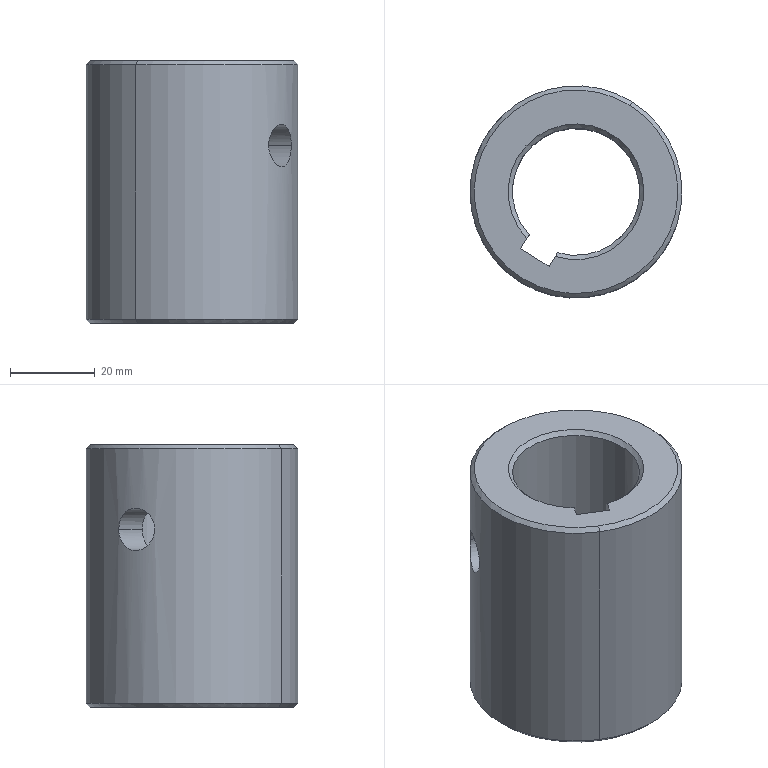Component | SolidWorks | 29-1 | 1 solid | 19 faces | box 50 x 50 x 62 mm | volume 74358 mm3 | cone 7 | cylinder 7 | plane 5 | commonest cylinder face diameters 10 x4 50 x2 30 x1
build123d program:
from build123d import *

# Parameters (mm, degrees)
SKETCH1_R           = 25
BOSS_EXTRUDE1_DEPTH = 31
SKETCH2_R           = 5
CUT_EXTRUDE1_DEPTH  = 31
CHAMFER1_SIZE       = 1
CHAMFER2_SIZE       = 1


with BuildPart() as part:
    # Sketch1 → Boss-Extrude1 (new, symmetric)
    with BuildSketch(Plane(origin=(0, 0, 0), x_dir=(1, 0, 0), z_dir=(0, 1, 0))):
        with Locations(Location((0, 0, 0), (0, 0, 270))):
            Circle(SKETCH1_R)
        with BuildLine():
            Line((4, 18.3), (-4, 18.3))
            Line((-4, 18.3), (-4, 14.457))
            ThreePointArc((-4, 14.457), (0, -15), (4, 14.457))
            Line((4, 14.457), (4, 18.3))
        make_face(mode=Mode.SUBTRACT)
    extrude(amount=BOSS_EXTRUDE1_DEPTH, both=True)

    # Sketch2 → Cut-Extrude1 (cut, symmetric)
    with BuildSketch(Plane(origin=(0, 0, 0), x_dir=(0, 0, -1), z_dir=(1, 0, 0))):
        with Locations((0, -11)):
            Circle(SKETCH2_R)
    extrude(amount=CUT_EXTRUDE1_DEPTH, both=True, mode=Mode.SUBTRACT)

    # Chamfer1
    chamfer1_edges = [part.edges().sort_by_distance(p)[0] for p in [
        (0, -31, 15),
        (0, 31, 15),
    ]]
    chamfer(chamfer1_edges, length=CHAMFER1_SIZE)

    # Chamfer2
    chamfer2_edges = [part.edges().sort_by_distance(p)[0] for p in [
        (0, -31, -25),
        (0, 31, -25),
    ]]
    chamfer(chamfer2_edges, length=CHAMFER2_SIZE)


solid = part.part

# Placed as in the assembly
solid = solid.moved(Location((70, -47, 137.06), (-89.999, 32.126, -0.0008769)))
STEP:
#1=CARTESIAN_POINT('',(2.253,-2.651,6.617));
#2=VERTEX_POINT('',#1);
#3=CARTESIAN_POINT('',(3.258,-1.05,6.617));
#4=VERTEX_POINT('',#3);
#5=CARTESIAN_POINT('',(2.756,-1.85,6.617));
#6=DIRECTION('',(0.,0.,1.));
#7=DIRECTION('',(0.5318,0.8469,0.));
#8=AXIS2_PLACEMENT_3D('',#5,#6,#7);
#9=CIRCLE('',#8,0.9449);
#10=EDGE_CURVE('',#2,#4,#9,.T.);
#11=ORIENTED_EDGE('',*,*,#10,.F.);
#12=CARTESIAN_POINT('',(2.232,-2.684,6.577));
#13=VERTEX_POINT('',#12);
#14=CARTESIAN_POINT('',(2.232,-2.684,6.577));
#15=DIRECTION('',(-0.376,-0.5988,-0.7071));
#16=VECTOR('',#15,39.37);
#17=LINE('',#14,#16);
#18=EDGE_CURVE('',#2,#13,#17,.T.);
#19=ORIENTED_EDGE('',*,*,#18,.T.);
#20=CARTESIAN_POINT('',(3.279,-1.017,6.577));
#21=VERTEX_POINT('',#20);
#22=CARTESIAN_POINT('',(2.756,-1.85,6.577));
#23=DIRECTION('',(-0.,-0.,-1.));
#24=DIRECTION('',(0.5318,0.8469,0.));
#25=AXIS2_PLACEMENT_3D('',#22,#23,#24);
#26=CIRCLE('',#25,0.9843);
#27=EDGE_CURVE('',#21,#13,#26,.T.);
#28=ORIENTED_EDGE('',*,*,#27,.F.);
#29=CARTESIAN_POINT('',(3.279,-1.017,6.577));
#30=DIRECTION('',(0.376,0.5988,-0.7071));
#31=VECTOR('',#30,39.37);
#32=LINE('',#29,#31);
#33=EDGE_CURVE('',#4,#21,#32,.T.);
#34=ORIENTED_EDGE('',*,*,#33,.F.);
#35=EDGE_LOOP('',(#11,#19,#28,#34));
#36=FACE_OUTER_BOUND('',#35,.T.);
#37=CARTESIAN_POINT('',(2.756,-1.85,6.577));
#38=DIRECTION('',(-0.,-0.,-1.));
#39=DIRECTION('',(0.5318,0.8469,0.));
#40=AXIS2_PLACEMENT_3D('',#37,#38,#39);
#41=CONICAL_SURFACE('',#40,0.9843,0.7854);
#42=ADVANCED_FACE('',(#36),#41,.T.);
#43=CARTESIAN_POINT('',(3.258,-1.05,4.176));
#44=VERTEX_POINT('',#43);
#45=CARTESIAN_POINT('',(2.253,-2.651,4.176));
#46=VERTEX_POINT('',#45);
#47=CARTESIAN_POINT('',(2.756,-1.85,4.176));
#48=DIRECTION('',(-0.,-0.,-1.));
#49=DIRECTION('',(0.5318,0.8469,0.));
#50=AXIS2_PLACEMENT_3D('',#47,#48,#49);
#51=CIRCLE('',#50,0.9449);
#52=EDGE_CURVE('',#44,#46,#51,.T.);
#53=ORIENTED_EDGE('',*,*,#52,.F.);
#54=CARTESIAN_POINT('',(3.279,-1.017,4.215));
#55=VERTEX_POINT('',#54);
#56=CARTESIAN_POINT('',(3.258,-1.05,4.176));
#57=DIRECTION('',(0.376,0.5988,0.7071));
#58=VECTOR('',#57,39.37);
#59=LINE('',#56,#58);
#60=EDGE_CURVE('',#44,#55,#59,.T.);
#61=ORIENTED_EDGE('',*,*,#60,.T.);
#62=CARTESIAN_POINT('',(2.232,-2.684,4.215));
#63=VERTEX_POINT('',#62);
#64=CARTESIAN_POINT('',(2.756,-1.85,4.215));
#65=DIRECTION('',(0.,0.,1.));
#66=DIRECTION('',(0.5318,0.8469,0.));
#67=AXIS2_PLACEMENT_3D('',#64,#65,#66);
#68=CIRCLE('',#67,0.9843);
#69=EDGE_CURVE('',#63,#55,#68,.T.);
#70=ORIENTED_EDGE('',*,*,#69,.F.);
#71=CARTESIAN_POINT('',(2.253,-2.651,4.176));
#72=DIRECTION('',(-0.376,-0.5988,0.7071));
#73=VECTOR('',#72,39.37);
#74=LINE('',#71,#73);
#75=EDGE_CURVE('',#46,#63,#74,.T.);
#76=ORIENTED_EDGE('',*,*,#75,.F.);
#77=EDGE_LOOP('',(#53,#61,#70,#76));
#78=FACE_OUTER_BOUND('',#77,.T.);
#79=CARTESIAN_POINT('',(2.756,-1.85,4.176));
#80=DIRECTION('',(0.,0.,1.));
#81=DIRECTION('',(-0.5318,-0.8469,0.));
#82=AXIS2_PLACEMENT_3D('',#79,#80,#81);
#83=CONICAL_SURFACE('',#82,0.9449,0.7854);
#84=ADVANCED_FACE('',(#78),#83,.T.);
#85=CARTESIAN_POINT('',(3.07,-1.35,4.215));
#86=VERTEX_POINT('',#85);
#87=CARTESIAN_POINT('',(2.587,-2.416,4.215));
#88=VERTEX_POINT('',#87);
#89=CARTESIAN_POINT('',(2.756,-1.85,4.215));
#90=DIRECTION('',(-0.,-0.,-1.));
#91=DIRECTION('',(0.5318,0.8469,0.));
#92=AXIS2_PLACEMENT_3D('',#89,#90,#91);
#93=CIRCLE('',#92,0.5906);
#94=EDGE_CURVE('',#86,#88,#93,.T.);
#95=ORIENTED_EDGE('',*,*,#94,.F.);
#96=CARTESIAN_POINT('',(3.091,-1.317,4.176));
#97=VERTEX_POINT('',#96);
#98=CARTESIAN_POINT('',(3.07,-1.35,4.215));
#99=DIRECTION('',(0.376,0.5988,-0.7071));
#100=VECTOR('',#99,39.37);
#101=LINE('',#98,#100);
#102=EDGE_CURVE('',#86,#97,#101,.T.);
#103=ORIENTED_EDGE('',*,*,#102,.T.);
#104=CARTESIAN_POINT('',(2.565,-2.451,4.176));
#105=VERTEX_POINT('',#104);
#106=CARTESIAN_POINT('',(2.756,-1.85,4.176));
#107=DIRECTION('',(0.,0.,1.));
#108=DIRECTION('',(0.5318,0.8469,0.));
#109=AXIS2_PLACEMENT_3D('',#106,#107,#108);
#110=CIRCLE('',#109,0.6299);
#111=EDGE_CURVE('',#105,#97,#110,.T.);
#112=ORIENTED_EDGE('',*,*,#111,.F.);
#113=CARTESIAN_POINT('',(2.587,-2.416,4.215));
#114=CARTESIAN_POINT('',(2.579,-2.428,4.202));
#115=CARTESIAN_POINT('',(2.572,-2.439,4.189));
#116=CARTESIAN_POINT('',(2.565,-2.451,4.176));
#117=B_SPLINE_CURVE_WITH_KNOTS('',3,(#113,#114,#115,#116),.UNSPECIFIED.,.F.,.F.,(4,4),(0.,0.001439),.UNSPECIFIED.);
#118=EDGE_CURVE('',#88,#105,#117,.T.);
#119=ORIENTED_EDGE('',*,*,#118,.F.);
#120=EDGE_LOOP('',(#95,#103,#112,#119));
#121=FACE_OUTER_BOUND('',#120,.T.);
#122=CARTESIAN_POINT('',(2.756,-1.85,4.215));
#123=DIRECTION('',(-0.,-0.,-1.));
#124=DIRECTION('',(0.5318,0.8469,0.));
#125=AXIS2_PLACEMENT_3D('',#122,#123,#124);
#126=CONICAL_SURFACE('',#125,0.5906,0.7854);
#127=ADVANCED_FACE('',(#121),#126,.F.);
#128=CARTESIAN_POINT('',(2.044,-1.171,5.829));
#129=VERTEX_POINT('',#128);
#130=CARTESIAN_POINT('',(1.835,-1.504,5.829));
#131=VERTEX_POINT('',#130);
#132=CARTESIAN_POINT('',(2.044,-1.171,5.829));
#133=CARTESIAN_POINT('',(2.044,-1.171,5.842));
#134=CARTESIAN_POINT('',(2.043,-1.172,5.855));
#135=CARTESIAN_POINT('',(2.039,-1.176,5.88));
#136=CARTESIAN_POINT('',(2.037,-1.178,5.893));
#137=CARTESIAN_POINT('',(2.032,-1.184,5.91));
#138=CARTESIAN_POINT('',(2.03,-1.186,5.916));
#139=CARTESIAN_POINT('',(2.026,-1.19,5.928));
#140=CARTESIAN_POINT('',(2.023,-1.193,5.933));
#141=CARTESIAN_POINT('',(2.016,-1.201,5.949));
#142=CARTESIAN_POINT('',(2.011,-1.207,5.959));
#143=CARTESIAN_POINT('',(1.999,-1.221,5.977));
#144=CARTESIAN_POINT('',(1.992,-1.229,5.986));
#145=CARTESIAN_POINT('',(1.979,-1.246,6.));
#146=CARTESIAN_POINT('',(1.972,-1.255,6.006));
#147=CARTESIAN_POINT('',(1.958,-1.274,6.016));
#148=CARTESIAN_POINT('',(1.951,-1.284,6.02));
#149=CARTESIAN_POINT('',(1.936,-1.305,6.025));
#150=CARTESIAN_POINT('',(1.929,-1.316,6.026));
#151=CARTESIAN_POINT('',(1.916,-1.338,6.026));
#152=CARTESIAN_POINT('',(1.909,-1.349,6.025));
#153=CARTESIAN_POINT('',(1.896,-1.371,6.02));
#154=CARTESIAN_POINT('',(1.89,-1.382,6.016));
#155=CARTESIAN_POINT('',(1.879,-1.403,6.006));
#156=CARTESIAN_POINT('',(1.874,-1.413,6.));
#157=CARTESIAN_POINT('',(1.867,-1.428,5.989));
#158=CARTESIAN_POINT('',(1.865,-1.432,5.985));
#159=CARTESIAN_POINT('',(1.861,-1.442,5.977));
#160=CARTESIAN_POINT('',(1.859,-1.446,5.973));
#161=CARTESIAN_POINT('',(1.853,-1.458,5.959));
#162=CARTESIAN_POINT('',(1.85,-1.466,5.949));
#163=CARTESIAN_POINT('',(1.844,-1.48,5.928));
#164=CARTESIAN_POINT('',(1.842,-1.485,5.917));
#165=CARTESIAN_POINT('',(1.838,-1.495,5.893));
#166=CARTESIAN_POINT('',(1.837,-1.498,5.88));
#167=CARTESIAN_POINT('',(1.835,-1.503,5.855));
#168=CARTESIAN_POINT('',(1.835,-1.504,5.842));
#169=CARTESIAN_POINT('',(1.835,-1.504,5.829));
#170=B_SPLINE_CURVE_WITH_KNOTS('',3,(#132,#133,#134,#135,#136,#137,#138,#139,#140,#141,#142,#143,#144,#145,#146,#147,#148,#149,#150,#151,#152,#153,#154,#155,#156,#157,#158,#159,#160,#161,#162,#163,#164,#165,#166,#167,#168,#169),.UNSPECIFIED.,.F.,.F.,(4,2,2,2,2,2,2,2,2,2,2,2,2,2,2,2,2,2,4),(0.01567,0.01665,0.01763,0.01812,0.01861,0.01959,0.02057,0.02155,0.02253,0.02351,0.02448,0.02546,0.02644,0.02693,0.02742,0.0284,0.02938,0.03036,0.03134),.UNSPECIFIED.);
#171=EDGE_CURVE('',#129,#131,#170,.T.);
#172=ORIENTED_EDGE('',*,*,#171,.F.);
#173=CARTESIAN_POINT('',(2.389,-1.388,5.829));
#174=VERTEX_POINT('',#173);
#175=CARTESIAN_POINT('',(1.827,-1.035,5.829));
#176=DIRECTION('',(0.8469,-0.5318,-0.));
#177=VECTOR('',#176,39.37);
#178=LINE('',#175,#177);
#179=EDGE_CURVE('',#129,#174,#178,.T.);
#180=ORIENTED_EDGE('',*,*,#179,.T.);
#181=CARTESIAN_POINT('',(2.18,-1.721,5.829));
#182=VERTEX_POINT('',#181);
#183=CARTESIAN_POINT('',(2.389,-1.388,5.829));
#184=CARTESIAN_POINT('',(2.389,-1.388,5.842));
#185=CARTESIAN_POINT('',(2.388,-1.388,5.855));
#186=CARTESIAN_POINT('',(2.384,-1.392,5.881));
#187=CARTESIAN_POINT('',(2.381,-1.394,5.893));
#188=CARTESIAN_POINT('',(2.373,-1.401,5.917));
#189=CARTESIAN_POINT('',(2.368,-1.405,5.928));
#190=CARTESIAN_POINT('',(2.357,-1.415,5.949));
#191=CARTESIAN_POINT('',(2.351,-1.421,5.959));
#192=CARTESIAN_POINT('',(2.337,-1.434,5.977));
#193=CARTESIAN_POINT('',(2.33,-1.441,5.986));
#194=CARTESIAN_POINT('',(2.315,-1.457,6.));
#195=CARTESIAN_POINT('',(2.308,-1.466,6.006));
#196=CARTESIAN_POINT('',(2.292,-1.484,6.016));
#197=CARTESIAN_POINT('',(2.285,-1.494,6.02));
#198=CARTESIAN_POINT('',(2.27,-1.514,6.025));
#199=CARTESIAN_POINT('',(2.263,-1.525,6.026));
#200=CARTESIAN_POINT('',(2.249,-1.547,6.026));
#201=CARTESIAN_POINT('',(2.242,-1.558,6.025));
#202=CARTESIAN_POINT('',(2.233,-1.575,6.021));
#203=CARTESIAN_POINT('',(2.23,-1.581,6.019));
#204=CARTESIAN_POINT('',(2.225,-1.592,6.016));
#205=CARTESIAN_POINT('',(2.222,-1.598,6.013));
#206=CARTESIAN_POINT('',(2.215,-1.614,6.006));
#207=CARTESIAN_POINT('',(2.21,-1.624,6.));
#208=CARTESIAN_POINT('',(2.202,-1.645,5.985));
#209=CARTESIAN_POINT('',(2.199,-1.654,5.977));
#210=CARTESIAN_POINT('',(2.193,-1.672,5.959));
#211=CARTESIAN_POINT('',(2.19,-1.68,5.949));
#212=CARTESIAN_POINT('',(2.186,-1.694,5.928));
#213=CARTESIAN_POINT('',(2.185,-1.7,5.917));
#214=CARTESIAN_POINT('',(2.182,-1.711,5.893));
#215=CARTESIAN_POINT('',(2.181,-1.714,5.88));
#216=CARTESIAN_POINT('',(2.18,-1.72,5.855));
#217=CARTESIAN_POINT('',(2.18,-1.721,5.842));
#218=CARTESIAN_POINT('',(2.18,-1.721,5.829));
#219=B_SPLINE_CURVE_WITH_KNOTS('',3,(#183,#184,#185,#186,#187,#188,#189,#190,#191,#192,#193,#194,#195,#196,#197,#198,#199,#200,#201,#202,#203,#204,#205,#206,#207,#208,#209,#210,#211,#212,#213,#214,#215,#216,#217,#218),.UNSPECIFIED.,.F.,.F.,(4,2,2,2,2,2,2,2,2,2,2,2,2,2,2,2,2,4),(0.01575,0.01673,0.01771,0.0187,0.01968,0.02066,0.02165,0.02263,0.02362,0.0246,0.02509,0.02558,0.02657,0.02755,0.02854,0.02952,0.0305,0.03149),.UNSPECIFIED.);
#220=EDGE_CURVE('',#174,#182,#219,.T.);
#221=ORIENTED_EDGE('',*,*,#220,.T.);
#222=CARTESIAN_POINT('',(1.618,-1.368,5.829));
#223=DIRECTION('',(0.8469,-0.5318,-0.));
#224=VECTOR('',#223,39.37);
#225=LINE('',#222,#224);
#226=EDGE_CURVE('',#131,#182,#225,.T.);
#227=ORIENTED_EDGE('',*,*,#226,.F.);
#228=EDGE_LOOP('',(#172,#180,#221,#227));
#229=FACE_OUTER_BOUND('',#228,.T.);
#230=CARTESIAN_POINT('',(1.722,-1.201,5.829));
#231=DIRECTION('',(0.8469,-0.5318,-0.));
#232=DIRECTION('',(-0.5318,-0.8469,0.));
#233=AXIS2_PLACEMENT_3D('',#230,#231,#232);
#234=CYLINDRICAL_SURFACE('',#233,0.1969);
#235=ADVANCED_FACE('',(#229),#234,.F.);
#236=CARTESIAN_POINT('',(3.123,-2.313,5.829));
#237=VERTEX_POINT('',#236);
#238=CARTESIAN_POINT('',(3.332,-1.98,5.829));
#239=VERTEX_POINT('',#238);
#240=CARTESIAN_POINT('',(3.123,-2.313,5.829));
#241=CARTESIAN_POINT('',(3.123,-2.313,5.842));
#242=CARTESIAN_POINT('',(3.124,-2.312,5.855));
#243=CARTESIAN_POINT('',(3.128,-2.309,5.88));
#244=CARTESIAN_POINT('',(3.131,-2.306,5.893));
#245=CARTESIAN_POINT('',(3.139,-2.3,5.917));
#246=CARTESIAN_POINT('',(3.144,-2.296,5.928));
#247=CARTESIAN_POINT('',(3.155,-2.286,5.949));
#248=CARTESIAN_POINT('',(3.161,-2.28,5.959));
#249=CARTESIAN_POINT('',(3.175,-2.267,5.977));
#250=CARTESIAN_POINT('',(3.182,-2.26,5.985));
#251=CARTESIAN_POINT('',(3.197,-2.244,6.));
#252=CARTESIAN_POINT('',(3.204,-2.235,6.006));
#253=CARTESIAN_POINT('',(3.215,-2.221,6.013));
#254=CARTESIAN_POINT('',(3.219,-2.217,6.015));
#255=CARTESIAN_POINT('',(3.227,-2.207,6.019));
#256=CARTESIAN_POINT('',(3.231,-2.202,6.021));
#257=CARTESIAN_POINT('',(3.242,-2.186,6.025));
#258=CARTESIAN_POINT('',(3.249,-2.175,6.026));
#259=CARTESIAN_POINT('',(3.263,-2.154,6.026));
#260=CARTESIAN_POINT('',(3.269,-2.142,6.025));
#261=CARTESIAN_POINT('',(3.282,-2.12,6.02));
#262=CARTESIAN_POINT('',(3.287,-2.109,6.016));
#263=CARTESIAN_POINT('',(3.297,-2.087,6.006));
#264=CARTESIAN_POINT('',(3.302,-2.076,6.));
#265=CARTESIAN_POINT('',(3.31,-2.056,5.986));
#266=CARTESIAN_POINT('',(3.313,-2.046,5.977));
#267=CARTESIAN_POINT('',(3.319,-2.029,5.959));
#268=CARTESIAN_POINT('',(3.321,-2.021,5.949));
#269=CARTESIAN_POINT('',(3.325,-2.007,5.928));
#270=CARTESIAN_POINT('',(3.327,-2.,5.917));
#271=CARTESIAN_POINT('',(3.33,-1.99,5.893));
#272=CARTESIAN_POINT('',(3.331,-1.986,5.881));
#273=CARTESIAN_POINT('',(3.332,-1.982,5.861));
#274=CARTESIAN_POINT('',(3.332,-1.981,5.855));
#275=CARTESIAN_POINT('',(3.332,-1.98,5.842));
#276=CARTESIAN_POINT('',(3.332,-1.98,5.836));
#277=CARTESIAN_POINT('',(3.332,-1.98,5.829));
#278=B_SPLINE_CURVE_WITH_KNOTS('',3,(#240,#241,#242,#243,#244,#245,#246,#247,#248,#249,#250,#251,#252,#253,#254,#255,#256,#257,#258,#259,#260,#261,#262,#263,#264,#265,#266,#267,#268,#269,#270,#271,#272,#273,#274,#275,#276,#277),.UNSPECIFIED.,.F.,.F.,(4,2,2,2,2,2,2,2,2,2,2,2,2,2,2,2,2,2,4),(0.,0.0009841,0.001968,0.002952,0.003936,0.00492,0.005905,0.006397,0.006889,0.007873,0.008857,0.009841,0.01082,0.01181,0.01279,0.01378,0.01476,0.01525,0.01575),.UNSPECIFIED.);
#279=EDGE_CURVE('',#237,#239,#278,.T.);
#280=ORIENTED_EDGE('',*,*,#279,.T.);
#281=CARTESIAN_POINT('',(3.677,-2.197,5.829));
#282=VERTEX_POINT('',#281);
#283=CARTESIAN_POINT('',(1.827,-1.035,5.829));
#284=DIRECTION('',(0.8469,-0.5318,-0.));
#285=VECTOR('',#284,39.37);
#286=LINE('',#283,#285);
#287=EDGE_CURVE('',#239,#282,#286,.T.);
#288=ORIENTED_EDGE('',*,*,#287,.T.);
#289=CARTESIAN_POINT('',(3.468,-2.53,5.829));
#290=VERTEX_POINT('',#289);
#291=CARTESIAN_POINT('',(3.468,-2.53,5.829));
#292=CARTESIAN_POINT('',(3.468,-2.53,5.842));
#293=CARTESIAN_POINT('',(3.469,-2.529,5.855));
#294=CARTESIAN_POINT('',(3.472,-2.525,5.88));
#295=CARTESIAN_POINT('',(3.475,-2.522,5.893));
#296=CARTESIAN_POINT('',(3.482,-2.515,5.917));
#297=CARTESIAN_POINT('',(3.486,-2.511,5.928));
#298=CARTESIAN_POINT('',(3.496,-2.5,5.949));
#299=CARTESIAN_POINT('',(3.501,-2.493,5.959));
#300=CARTESIAN_POINT('',(3.513,-2.479,5.977));
#301=CARTESIAN_POINT('',(3.519,-2.472,5.986));
#302=CARTESIAN_POINT('',(3.533,-2.455,6.));
#303=CARTESIAN_POINT('',(3.54,-2.446,6.006));
#304=CARTESIAN_POINT('',(3.554,-2.427,6.016));
#305=CARTESIAN_POINT('',(3.561,-2.416,6.02));
#306=CARTESIAN_POINT('',(3.576,-2.395,6.025));
#307=CARTESIAN_POINT('',(3.583,-2.385,6.026));
#308=CARTESIAN_POINT('',(3.596,-2.363,6.026));
#309=CARTESIAN_POINT('',(3.603,-2.352,6.025));
#310=CARTESIAN_POINT('',(3.616,-2.33,6.02));
#311=CARTESIAN_POINT('',(3.622,-2.319,6.016));
#312=CARTESIAN_POINT('',(3.63,-2.303,6.008));
#313=CARTESIAN_POINT('',(3.633,-2.298,6.006));
#314=CARTESIAN_POINT('',(3.638,-2.288,6.));
#315=CARTESIAN_POINT('',(3.64,-2.283,5.996));
#316=CARTESIAN_POINT('',(3.647,-2.268,5.986));
#317=CARTESIAN_POINT('',(3.651,-2.259,5.977));
#318=CARTESIAN_POINT('',(3.659,-2.242,5.959));
#319=CARTESIAN_POINT('',(3.662,-2.235,5.949));
#320=CARTESIAN_POINT('',(3.668,-2.221,5.928));
#321=CARTESIAN_POINT('',(3.67,-2.215,5.916));
#322=CARTESIAN_POINT('',(3.674,-2.206,5.893));
#323=CARTESIAN_POINT('',(3.675,-2.203,5.88));
#324=CARTESIAN_POINT('',(3.677,-2.198,5.855));
#325=CARTESIAN_POINT('',(3.677,-2.197,5.842));
#326=CARTESIAN_POINT('',(3.677,-2.197,5.829));
#327=B_SPLINE_CURVE_WITH_KNOTS('',3,(#291,#292,#293,#294,#295,#296,#297,#298,#299,#300,#301,#302,#303,#304,#305,#306,#307,#308,#309,#310,#311,#312,#313,#314,#315,#316,#317,#318,#319,#320,#321,#322,#323,#324,#325,#326),.UNSPECIFIED.,.F.,.F.,(4,2,2,2,2,2,2,2,2,2,2,2,2,2,2,2,2,4),(0.,0.0009795,0.001959,0.002938,0.003918,0.004897,0.005877,0.006856,0.007836,0.008815,0.009795,0.01028,0.01077,0.01175,0.01273,0.01371,0.01469,0.01567),.UNSPECIFIED.);
#328=EDGE_CURVE('',#290,#282,#327,.T.);
#329=ORIENTED_EDGE('',*,*,#328,.F.);
#330=CARTESIAN_POINT('',(1.618,-1.368,5.829));
#331=DIRECTION('',(0.8469,-0.5318,-0.));
#332=VECTOR('',#331,39.37);
#333=LINE('',#330,#332);
#334=EDGE_CURVE('',#237,#290,#333,.T.);
#335=ORIENTED_EDGE('',*,*,#334,.F.);
#336=EDGE_LOOP('',(#280,#288,#329,#335));
#337=FACE_OUTER_BOUND('',#336,.T.);
#338=CARTESIAN_POINT('',(1.722,-1.201,5.829));
#339=DIRECTION('',(0.8469,-0.5318,-0.));
#340=DIRECTION('',(-0.5318,-0.8469,0.));
#341=AXIS2_PLACEMENT_3D('',#338,#339,#340);
#342=CYLINDRICAL_SURFACE('',#341,0.1969);
#343=ADVANCED_FACE('',(#337),#342,.F.);
#344=ORIENTED_EDGE('',*,*,#328,.T.);
#345=CARTESIAN_POINT('',(3.677,-2.197,5.829));
#346=CARTESIAN_POINT('',(3.677,-2.197,5.816));
#347=CARTESIAN_POINT('',(3.677,-2.198,5.803));
#348=CARTESIAN_POINT('',(3.675,-2.203,5.778));
#349=CARTESIAN_POINT('',(3.674,-2.206,5.766));
#350=CARTESIAN_POINT('',(3.671,-2.213,5.748));
#351=CARTESIAN_POINT('',(3.67,-2.216,5.742));
#352=CARTESIAN_POINT('',(3.668,-2.221,5.731));
#353=CARTESIAN_POINT('',(3.666,-2.225,5.725));
#354=CARTESIAN_POINT('',(3.662,-2.235,5.709));
#355=CARTESIAN_POINT('',(3.659,-2.242,5.699));
#356=CARTESIAN_POINT('',(3.651,-2.259,5.681));
#357=CARTESIAN_POINT('',(3.647,-2.268,5.673));
#358=CARTESIAN_POINT('',(3.638,-2.288,5.658));
#359=CARTESIAN_POINT('',(3.633,-2.298,5.652));
#360=CARTESIAN_POINT('',(3.622,-2.319,5.642));
#361=CARTESIAN_POINT('',(3.616,-2.33,5.639));
#362=CARTESIAN_POINT('',(3.603,-2.352,5.634));
#363=CARTESIAN_POINT('',(3.596,-2.363,5.632));
#364=CARTESIAN_POINT('',(3.583,-2.385,5.632));
#365=CARTESIAN_POINT('',(3.576,-2.395,5.634));
#366=CARTESIAN_POINT('',(3.561,-2.416,5.639));
#367=CARTESIAN_POINT('',(3.554,-2.427,5.642));
#368=CARTESIAN_POINT('',(3.54,-2.446,5.652));
#369=CARTESIAN_POINT('',(3.533,-2.455,5.658));
#370=CARTESIAN_POINT('',(3.523,-2.467,5.669));
#371=CARTESIAN_POINT('',(3.52,-2.471,5.673));
#372=CARTESIAN_POINT('',(3.513,-2.479,5.681));
#373=CARTESIAN_POINT('',(3.51,-2.483,5.685));
#374=CARTESIAN_POINT('',(3.501,-2.493,5.699));
#375=CARTESIAN_POINT('',(3.496,-2.5,5.709));
#376=CARTESIAN_POINT('',(3.486,-2.51,5.73));
#377=CARTESIAN_POINT('',(3.482,-2.515,5.742));
#378=CARTESIAN_POINT('',(3.475,-2.522,5.765));
#379=CARTESIAN_POINT('',(3.472,-2.525,5.778));
#380=CARTESIAN_POINT('',(3.469,-2.529,5.803));
#381=CARTESIAN_POINT('',(3.468,-2.53,5.816));
#382=CARTESIAN_POINT('',(3.468,-2.53,5.829));
#383=B_SPLINE_CURVE_WITH_KNOTS('',3,(#345,#346,#347,#348,#349,#350,#351,#352,#353,#354,#355,#356,#357,#358,#359,#360,#361,#362,#363,#364,#365,#366,#367,#368,#369,#370,#371,#372,#373,#374,#375,#376,#377,#378,#379,#380,#381,#382),.UNSPECIFIED.,.F.,.F.,(4,2,2,2,2,2,2,2,2,2,2,2,2,2,2,2,2,2,4),(0.01567,0.01665,0.01763,0.01812,0.01861,0.01959,0.02057,0.02155,0.02253,0.02351,0.02448,0.02546,0.02644,0.02693,0.02742,0.0284,0.02938,0.03036,0.03134),.UNSPECIFIED.);
#384=EDGE_CURVE('',#282,#290,#383,.T.);
#385=ORIENTED_EDGE('',*,*,#384,.T.);
#386=EDGE_LOOP('',(#344,#385));
#387=FACE_BOUND('',#386,.T.);
#388=ORIENTED_EDGE('',*,*,#69,.T.);
#389=CARTESIAN_POINT('',(3.279,-1.017,4.176));
#390=DIRECTION('',(0.,0.,1.));
#391=VECTOR('',#390,39.37);
#392=LINE('',#389,#391);
#393=EDGE_CURVE('',#55,#21,#392,.T.);
#394=ORIENTED_EDGE('',*,*,#393,.T.);
#395=ORIENTED_EDGE('',*,*,#27,.T.);
#396=CARTESIAN_POINT('',(2.232,-2.684,4.176));
#397=DIRECTION('',(0.,0.,1.));
#398=VECTOR('',#397,39.37);
#399=LINE('',#396,#398);
#400=EDGE_CURVE('',#63,#13,#399,.T.);
#401=ORIENTED_EDGE('',*,*,#400,.F.);
#402=EDGE_LOOP('',(#388,#394,#395,#401));
#403=FACE_OUTER_BOUND('',#402,.T.);
#404=CARTESIAN_POINT('',(2.756,-1.85,4.176));
#405=DIRECTION('',(0.,0.,1.));
#406=DIRECTION('',(-0.5318,-0.8469,0.));
#407=AXIS2_PLACEMENT_3D('',#404,#405,#406);
#408=CYLINDRICAL_SURFACE('',#407,0.9843);
#409=ADVANCED_FACE('',(#387,#403),#408,.T.);
#410=CARTESIAN_POINT('',(2.756,-1.85,4.176));
#411=DIRECTION('',(-0.,-0.,-1.));
#412=DIRECTION('',(0.5318,0.8469,0.));
#413=AXIS2_PLACEMENT_3D('',#410,#411,#412);
#414=CIRCLE('',#413,0.9449);
#415=EDGE_CURVE('',#46,#44,#414,.T.);
#416=ORIENTED_EDGE('',*,*,#415,.T.);
#417=ORIENTED_EDGE('',*,*,#52,.T.);
#418=EDGE_LOOP('',(#416,#417));
#419=FACE_OUTER_BOUND('',#418,.T.);
#420=CARTESIAN_POINT('',(2.506,-2.544,4.176));
#421=VERTEX_POINT('',#420);
#422=CARTESIAN_POINT('',(2.506,-2.544,4.176));
#423=DIRECTION('',(-0.5318,-0.8469,0.));
#424=VECTOR('',#423,39.37);
#425=LINE('',#422,#424);
#426=EDGE_CURVE('',#105,#421,#425,.T.);
#427=ORIENTED_EDGE('',*,*,#426,.F.);
#428=ORIENTED_EDGE('',*,*,#111,.T.);
#429=CARTESIAN_POINT('',(2.298,-2.283,4.176));
#430=VERTEX_POINT('',#429);
#431=CARTESIAN_POINT('',(2.756,-1.85,4.176));
#432=DIRECTION('',(0.,0.,1.));
#433=DIRECTION('',(0.5318,0.8469,0.));
#434=AXIS2_PLACEMENT_3D('',#431,#432,#433);
#435=CIRCLE('',#434,0.6299);
#436=EDGE_CURVE('',#97,#430,#435,.T.);
#437=ORIENTED_EDGE('',*,*,#436,.T.);
#438=CARTESIAN_POINT('',(2.239,-2.377,4.176));
#439=VERTEX_POINT('',#438);
#440=CARTESIAN_POINT('',(2.239,-2.377,4.176));
#441=DIRECTION('',(0.5318,0.8469,-0.));
#442=VECTOR('',#441,39.37);
#443=LINE('',#440,#442);
#444=EDGE_CURVE('',#439,#430,#443,.T.);
#445=ORIENTED_EDGE('',*,*,#444,.F.);
#446=CARTESIAN_POINT('',(2.506,-2.544,4.176));
#447=DIRECTION('',(-0.8469,0.5318,0.));
#448=VECTOR('',#447,39.37);
#449=LINE('',#446,#448);
#450=EDGE_CURVE('',#421,#439,#449,.T.);
#451=ORIENTED_EDGE('',*,*,#450,.F.);
#452=EDGE_LOOP('',(#427,#428,#437,#445,#451));
#453=FACE_BOUND('',#452,.T.);
#454=CARTESIAN_POINT('',(2.756,-1.85,4.176));
#455=DIRECTION('',(-0.,-0.,-1.));
#456=DIRECTION('',(0.5318,0.8469,-0.));
#457=AXIS2_PLACEMENT_3D('',#454,#455,#456);
#458=PLANE('',#457);
#459=ADVANCED_FACE('',(#419,#453),#458,.T.);
#460=CARTESIAN_POINT('',(2.756,-1.85,6.617));
#461=DIRECTION('',(0.,0.,1.));
#462=DIRECTION('',(0.5318,0.8469,0.));
#463=AXIS2_PLACEMENT_3D('',#460,#461,#462);
#464=CIRCLE('',#463,0.9449);
#465=EDGE_CURVE('',#4,#2,#464,.T.);
#466=ORIENTED_EDGE('',*,*,#465,.T.);
#467=ORIENTED_EDGE('',*,*,#10,.T.);
#468=EDGE_LOOP('',(#466,#467));
#469=FACE_OUTER_BOUND('',#468,.T.);
#470=CARTESIAN_POINT('',(2.239,-2.377,6.617));
#471=VERTEX_POINT('',#470);
#472=CARTESIAN_POINT('',(2.298,-2.283,6.617));
#473=VERTEX_POINT('',#472);
#474=CARTESIAN_POINT('',(2.239,-2.377,6.617));
#475=DIRECTION('',(0.5318,0.8469,-0.));
#476=VECTOR('',#475,39.37);
#477=LINE('',#474,#476);
#478=EDGE_CURVE('',#471,#473,#477,.T.);
#479=ORIENTED_EDGE('',*,*,#478,.T.);
#480=CARTESIAN_POINT('',(2.565,-2.451,6.617));
#481=VERTEX_POINT('',#480);
#482=CARTESIAN_POINT('',(2.756,-1.85,6.617));
#483=DIRECTION('',(-0.,-0.,-1.));
#484=DIRECTION('',(0.5318,0.8469,0.));
#485=AXIS2_PLACEMENT_3D('',#482,#483,#484);
#486=CIRCLE('',#485,0.6299);
#487=EDGE_CURVE('',#473,#481,#486,.T.);
#488=ORIENTED_EDGE('',*,*,#487,.T.);
#489=CARTESIAN_POINT('',(2.506,-2.544,6.617));
#490=VERTEX_POINT('',#489);
#491=CARTESIAN_POINT('',(2.506,-2.544,6.617));
#492=DIRECTION('',(-0.5318,-0.8469,0.));
#493=VECTOR('',#492,39.37);
#494=LINE('',#491,#493);
#495=EDGE_CURVE('',#481,#490,#494,.T.);
#496=ORIENTED_EDGE('',*,*,#495,.T.);
#497=CARTESIAN_POINT('',(2.506,-2.544,6.617));
#498=DIRECTION('',(-0.8469,0.5318,0.));
#499=VECTOR('',#498,39.37);
#500=LINE('',#497,#499);
#501=EDGE_CURVE('',#490,#471,#500,.T.);
#502=ORIENTED_EDGE('',*,*,#501,.T.);
#503=EDGE_LOOP('',(#479,#488,#496,#502));
#504=FACE_BOUND('',#503,.T.);
#505=CARTESIAN_POINT('',(2.756,-1.85,6.617));
#506=DIRECTION('',(-0.,-0.,-1.));
#507=DIRECTION('',(0.5318,0.8469,-0.));
#508=AXIS2_PLACEMENT_3D('',#505,#506,#507);
#509=PLANE('',#508);
#510=ADVANCED_FACE('',(#469,#504),#509,.F.);
#511=ORIENTED_EDGE('',*,*,#393,.F.);
#512=CARTESIAN_POINT('',(2.756,-1.85,4.215));
#513=DIRECTION('',(0.,0.,1.));
#514=DIRECTION('',(0.5318,0.8469,0.));
#515=AXIS2_PLACEMENT_3D('',#512,#513,#514);
#516=CIRCLE('',#515,0.9843);
#517=EDGE_CURVE('',#55,#63,#516,.T.);
#518=ORIENTED_EDGE('',*,*,#517,.T.);
#519=ORIENTED_EDGE('',*,*,#400,.T.);
#520=CARTESIAN_POINT('',(2.756,-1.85,6.577));
#521=DIRECTION('',(-0.,-0.,-1.));
#522=DIRECTION('',(0.5318,0.8469,0.));
#523=AXIS2_PLACEMENT_3D('',#520,#521,#522);
#524=CIRCLE('',#523,0.9843);
#525=EDGE_CURVE('',#13,#21,#524,.T.);
#526=ORIENTED_EDGE('',*,*,#525,.T.);
#527=EDGE_LOOP('',(#511,#518,#519,#526));
#528=FACE_OUTER_BOUND('',#527,.T.);
#529=CARTESIAN_POINT('',(1.835,-1.504,5.829));
#530=CARTESIAN_POINT('',(1.835,-1.504,5.816));
#531=CARTESIAN_POINT('',(1.835,-1.503,5.803));
#532=CARTESIAN_POINT('',(1.837,-1.498,5.778));
#533=CARTESIAN_POINT('',(1.838,-1.495,5.766));
#534=CARTESIAN_POINT('',(1.842,-1.485,5.742));
#535=CARTESIAN_POINT('',(1.844,-1.48,5.73));
#536=CARTESIAN_POINT('',(1.85,-1.466,5.709));
#537=CARTESIAN_POINT('',(1.853,-1.458,5.699));
#538=CARTESIAN_POINT('',(1.86,-1.442,5.681));
#539=CARTESIAN_POINT('',(1.865,-1.433,5.673));
#540=CARTESIAN_POINT('',(1.874,-1.413,5.658));
#541=CARTESIAN_POINT('',(1.879,-1.403,5.652));
#542=CARTESIAN_POINT('',(1.89,-1.382,5.642));
#543=CARTESIAN_POINT('',(1.896,-1.371,5.639));
#544=CARTESIAN_POINT('',(1.909,-1.349,5.634));
#545=CARTESIAN_POINT('',(1.915,-1.338,5.632));
#546=CARTESIAN_POINT('',(1.929,-1.316,5.632));
#547=CARTESIAN_POINT('',(1.936,-1.305,5.634));
#548=CARTESIAN_POINT('',(1.951,-1.284,5.639));
#549=CARTESIAN_POINT('',(1.958,-1.274,5.642));
#550=CARTESIAN_POINT('',(1.968,-1.26,5.65));
#551=CARTESIAN_POINT('',(1.972,-1.255,5.653));
#552=CARTESIAN_POINT('',(1.979,-1.246,5.659));
#553=CARTESIAN_POINT('',(1.982,-1.242,5.662));
#554=CARTESIAN_POINT('',(1.992,-1.229,5.673));
#555=CARTESIAN_POINT('',(1.999,-1.221,5.681));
#556=CARTESIAN_POINT('',(2.011,-1.207,5.699));
#557=CARTESIAN_POINT('',(2.016,-1.201,5.709));
#558=CARTESIAN_POINT('',(2.026,-1.19,5.73));
#559=CARTESIAN_POINT('',(2.03,-1.186,5.742));
#560=CARTESIAN_POINT('',(2.037,-1.178,5.766));
#561=CARTESIAN_POINT('',(2.039,-1.176,5.778));
#562=CARTESIAN_POINT('',(2.043,-1.172,5.803));
#563=CARTESIAN_POINT('',(2.044,-1.171,5.816));
#564=CARTESIAN_POINT('',(2.044,-1.171,5.829));
#565=B_SPLINE_CURVE_WITH_KNOTS('',3,(#529,#530,#531,#532,#533,#534,#535,#536,#537,#538,#539,#540,#541,#542,#543,#544,#545,#546,#547,#548,#549,#550,#551,#552,#553,#554,#555,#556,#557,#558,#559,#560,#561,#562,#563,#564),.UNSPECIFIED.,.F.,.F.,(4,2,2,2,2,2,2,2,2,2,2,2,2,2,2,2,2,4),(0.,0.0009795,0.001959,0.002938,0.003918,0.004897,0.005877,0.006856,0.007836,0.008815,0.009795,0.01028,0.01077,0.01175,0.01273,0.01371,0.01469,0.01567),.UNSPECIFIED.);
#566=EDGE_CURVE('',#131,#129,#565,.T.);
#567=ORIENTED_EDGE('',*,*,#566,.T.);
#568=ORIENTED_EDGE('',*,*,#171,.T.);
#569=EDGE_LOOP('',(#567,#568));
#570=FACE_BOUND('',#569,.T.);
#571=CARTESIAN_POINT('',(2.756,-1.85,4.176));
#572=DIRECTION('',(0.,0.,1.));
#573=DIRECTION('',(-0.5318,-0.8469,0.));
#574=AXIS2_PLACEMENT_3D('',#571,#572,#573);
#575=CYLINDRICAL_SURFACE('',#574,0.9843);
#576=ADVANCED_FACE('',(#528,#570),#575,.T.);
#577=CARTESIAN_POINT('',(2.32,-2.249,4.215));
#578=VERTEX_POINT('',#577);
#579=CARTESIAN_POINT('',(2.32,-2.249,6.577));
#580=VERTEX_POINT('',#579);
#581=CARTESIAN_POINT('',(2.32,-2.249,4.176));
#582=DIRECTION('',(0.,0.,1.));
#583=VECTOR('',#582,39.37);
#584=LINE('',#581,#583);
#585=EDGE_CURVE('',#578,#580,#584,.T.);
#586=ORIENTED_EDGE('',*,*,#585,.T.);
#587=CARTESIAN_POINT('',(2.32,-2.249,6.577));
#588=CARTESIAN_POINT('',(2.313,-2.26,6.59));
#589=CARTESIAN_POINT('',(2.305,-2.272,6.603));
#590=CARTESIAN_POINT('',(2.298,-2.283,6.617));
#591=B_SPLINE_CURVE_WITH_KNOTS('',3,(#587,#588,#589,#590),.UNSPECIFIED.,.F.,.F.,(4,4),(0.,0.001439),.UNSPECIFIED.);
#592=EDGE_CURVE('',#580,#473,#591,.T.);
#593=ORIENTED_EDGE('',*,*,#592,.T.);
#594=ORIENTED_EDGE('',*,*,#478,.F.);
#595=CARTESIAN_POINT('',(2.239,-2.377,4.176));
#596=DIRECTION('',(0.,0.,1.));
#597=VECTOR('',#596,39.37);
#598=LINE('',#595,#597);
#599=EDGE_CURVE('',#439,#471,#598,.T.);
#600=ORIENTED_EDGE('',*,*,#599,.F.);
#601=ORIENTED_EDGE('',*,*,#444,.T.);
#602=CARTESIAN_POINT('',(2.298,-2.283,4.176));
#603=CARTESIAN_POINT('',(2.305,-2.272,4.189));
#604=CARTESIAN_POINT('',(2.313,-2.26,4.202));
#605=CARTESIAN_POINT('',(2.32,-2.249,4.215));
#606=B_SPLINE_CURVE_WITH_KNOTS('',3,(#602,#603,#604,#605),.UNSPECIFIED.,.F.,.F.,(4,4),(0.,0.001439),.UNSPECIFIED.);
#607=EDGE_CURVE('',#430,#578,#606,.T.);
#608=ORIENTED_EDGE('',*,*,#607,.T.);
#609=EDGE_LOOP('',(#586,#593,#594,#600,#601,#608));
#610=FACE_OUTER_BOUND('',#609,.T.);
#611=CARTESIAN_POINT('',(2.239,-2.377,4.176));
#612=DIRECTION('',(0.8469,-0.5318,-0.));
#613=DIRECTION('',(-0.5318,-0.8469,0.));
#614=AXIS2_PLACEMENT_3D('',#611,#612,#613);
#615=PLANE('',#614);
#616=ADVANCED_FACE('',(#610),#615,.T.);
#617=CARTESIAN_POINT('',(2.18,-1.721,5.829));
#618=CARTESIAN_POINT('',(2.18,-1.721,5.816));
#619=CARTESIAN_POINT('',(2.18,-1.72,5.803));
#620=CARTESIAN_POINT('',(2.181,-1.714,5.778));
#621=CARTESIAN_POINT('',(2.182,-1.711,5.765));
#622=CARTESIAN_POINT('',(2.185,-1.7,5.742));
#623=CARTESIAN_POINT('',(2.186,-1.694,5.73));
#624=CARTESIAN_POINT('',(2.19,-1.68,5.709));
#625=CARTESIAN_POINT('',(2.193,-1.672,5.699));
#626=CARTESIAN_POINT('',(2.199,-1.654,5.681));
#627=CARTESIAN_POINT('',(2.202,-1.645,5.673));
#628=CARTESIAN_POINT('',(2.21,-1.624,5.658));
#629=CARTESIAN_POINT('',(2.215,-1.614,5.652));
#630=CARTESIAN_POINT('',(2.222,-1.598,5.645));
#631=CARTESIAN_POINT('',(2.225,-1.592,5.643));
#632=CARTESIAN_POINT('',(2.23,-1.581,5.639));
#633=CARTESIAN_POINT('',(2.233,-1.575,5.637));
#634=CARTESIAN_POINT('',(2.242,-1.558,5.634));
#635=CARTESIAN_POINT('',(2.249,-1.547,5.632));
#636=CARTESIAN_POINT('',(2.263,-1.525,5.632));
#637=CARTESIAN_POINT('',(2.27,-1.515,5.634));
#638=CARTESIAN_POINT('',(2.285,-1.494,5.639));
#639=CARTESIAN_POINT('',(2.292,-1.484,5.642));
#640=CARTESIAN_POINT('',(2.308,-1.466,5.652));
#641=CARTESIAN_POINT('',(2.315,-1.457,5.658));
#642=CARTESIAN_POINT('',(2.33,-1.441,5.673));
#643=CARTESIAN_POINT('',(2.337,-1.434,5.681));
#644=CARTESIAN_POINT('',(2.351,-1.421,5.699));
#645=CARTESIAN_POINT('',(2.357,-1.415,5.709));
#646=CARTESIAN_POINT('',(2.368,-1.405,5.73));
#647=CARTESIAN_POINT('',(2.373,-1.401,5.742));
#648=CARTESIAN_POINT('',(2.381,-1.394,5.765));
#649=CARTESIAN_POINT('',(2.384,-1.392,5.778));
#650=CARTESIAN_POINT('',(2.387,-1.389,5.797));
#651=CARTESIAN_POINT('',(2.388,-1.389,5.803));
#652=CARTESIAN_POINT('',(2.389,-1.388,5.816));
#653=CARTESIAN_POINT('',(2.389,-1.388,5.823));
#654=CARTESIAN_POINT('',(2.389,-1.388,5.829));
#655=B_SPLINE_CURVE_WITH_KNOTS('',3,(#617,#618,#619,#620,#621,#622,#623,#624,#625,#626,#627,#628,#629,#630,#631,#632,#633,#634,#635,#636,#637,#638,#639,#640,#641,#642,#643,#644,#645,#646,#647,#648,#649,#650,#651,#652,#653,#654),.UNSPECIFIED.,.F.,.F.,(4,2,2,2,2,2,2,2,2,2,2,2,2,2,2,2,2,2,4),(0.,0.0009841,0.001968,0.002952,0.003936,0.00492,0.005905,0.006397,0.006889,0.007873,0.008857,0.009841,0.01082,0.01181,0.01279,0.01378,0.01476,0.01525,0.01575),.UNSPECIFIED.);
#656=EDGE_CURVE('',#182,#174,#655,.T.);
#657=ORIENTED_EDGE('',*,*,#656,.F.);
#658=ORIENTED_EDGE('',*,*,#220,.F.);
#659=EDGE_LOOP('',(#657,#658));
#660=FACE_BOUND('',#659,.T.);
#661=ORIENTED_EDGE('',*,*,#279,.F.);
#662=CARTESIAN_POINT('',(3.332,-1.98,5.829));
#663=CARTESIAN_POINT('',(3.332,-1.98,5.816));
#664=CARTESIAN_POINT('',(3.332,-1.981,5.803));
#665=CARTESIAN_POINT('',(3.331,-1.986,5.778));
#666=CARTESIAN_POINT('',(3.33,-1.99,5.765));
#667=CARTESIAN_POINT('',(3.327,-2.,5.742));
#668=CARTESIAN_POINT('',(3.325,-2.007,5.73));
#669=CARTESIAN_POINT('',(3.321,-2.021,5.709));
#670=CARTESIAN_POINT('',(3.319,-2.029,5.699));
#671=CARTESIAN_POINT('',(3.313,-2.047,5.681));
#672=CARTESIAN_POINT('',(3.31,-2.056,5.673));
#673=CARTESIAN_POINT('',(3.302,-2.076,5.658));
#674=CARTESIAN_POINT('',(3.297,-2.087,5.652));
#675=CARTESIAN_POINT('',(3.287,-2.109,5.642));
#676=CARTESIAN_POINT('',(3.282,-2.12,5.639));
#677=CARTESIAN_POINT('',(3.27,-2.142,5.634));
#678=CARTESIAN_POINT('',(3.263,-2.153,5.632));
#679=CARTESIAN_POINT('',(3.249,-2.175,5.632));
#680=CARTESIAN_POINT('',(3.242,-2.186,5.634));
#681=CARTESIAN_POINT('',(3.231,-2.202,5.637));
#682=CARTESIAN_POINT('',(3.227,-2.207,5.639));
#683=CARTESIAN_POINT('',(3.219,-2.217,5.643));
#684=CARTESIAN_POINT('',(3.215,-2.221,5.645));
#685=CARTESIAN_POINT('',(3.204,-2.235,5.652));
#686=CARTESIAN_POINT('',(3.196,-2.244,5.658));
#687=CARTESIAN_POINT('',(3.182,-2.26,5.673));
#688=CARTESIAN_POINT('',(3.175,-2.267,5.681));
#689=CARTESIAN_POINT('',(3.161,-2.28,5.699));
#690=CARTESIAN_POINT('',(3.155,-2.286,5.709));
#691=CARTESIAN_POINT('',(3.144,-2.296,5.73));
#692=CARTESIAN_POINT('',(3.139,-2.3,5.742));
#693=CARTESIAN_POINT('',(3.131,-2.306,5.765));
#694=CARTESIAN_POINT('',(3.128,-2.309,5.778));
#695=CARTESIAN_POINT('',(3.124,-2.312,5.803));
#696=CARTESIAN_POINT('',(3.123,-2.313,5.816));
#697=CARTESIAN_POINT('',(3.123,-2.313,5.829));
#698=B_SPLINE_CURVE_WITH_KNOTS('',3,(#662,#663,#664,#665,#666,#667,#668,#669,#670,#671,#672,#673,#674,#675,#676,#677,#678,#679,#680,#681,#682,#683,#684,#685,#686,#687,#688,#689,#690,#691,#692,#693,#694,#695,#696,#697),.UNSPECIFIED.,.F.,.F.,(4,2,2,2,2,2,2,2,2,2,2,2,2,2,2,2,2,4),(0.01575,0.01673,0.01771,0.0187,0.01968,0.02066,0.02165,0.02263,0.02362,0.0246,0.02509,0.02558,0.02657,0.02755,0.02854,0.02952,0.0305,0.03149),.UNSPECIFIED.);
#699=EDGE_CURVE('',#239,#237,#698,.T.);
#700=ORIENTED_EDGE('',*,*,#699,.F.);
#701=EDGE_LOOP('',(#661,#700));
#702=FACE_BOUND('',#701,.T.);
#703=CARTESIAN_POINT('',(2.587,-2.416,6.577));
#704=VERTEX_POINT('',#703);
#705=CARTESIAN_POINT('',(2.587,-2.416,4.176));
#706=DIRECTION('',(0.,0.,1.));
#707=VECTOR('',#706,39.37);
#708=LINE('',#705,#707);
#709=EDGE_CURVE('',#88,#704,#708,.T.);
#710=ORIENTED_EDGE('',*,*,#709,.T.);
#711=CARTESIAN_POINT('',(2.756,-1.85,6.577));
#712=DIRECTION('',(0.,0.,1.));
#713=DIRECTION('',(0.5318,0.8469,0.));
#714=AXIS2_PLACEMENT_3D('',#711,#712,#713);
#715=CIRCLE('',#714,0.5906);
#716=EDGE_CURVE('',#704,#580,#715,.T.);
#717=ORIENTED_EDGE('',*,*,#716,.T.);
#718=ORIENTED_EDGE('',*,*,#585,.F.);
#719=CARTESIAN_POINT('',(2.756,-1.85,4.215));
#720=DIRECTION('',(-0.,-0.,-1.));
#721=DIRECTION('',(0.5318,0.8469,0.));
#722=AXIS2_PLACEMENT_3D('',#719,#720,#721);
#723=CIRCLE('',#722,0.5906);
#724=EDGE_CURVE('',#578,#86,#723,.T.);
#725=ORIENTED_EDGE('',*,*,#724,.T.);
#726=ORIENTED_EDGE('',*,*,#94,.T.);
#727=EDGE_LOOP('',(#710,#717,#718,#725,#726));
#728=FACE_OUTER_BOUND('',#727,.T.);
#729=CARTESIAN_POINT('',(2.756,-1.85,4.176));
#730=DIRECTION('',(0.,0.,1.));
#731=DIRECTION('',(-0.5318,-0.8469,0.));
#732=AXIS2_PLACEMENT_3D('',#729,#730,#731);
#733=CYLINDRICAL_SURFACE('',#732,0.5906);
#734=ADVANCED_FACE('',(#660,#702,#728),#733,.F.);
#735=ORIENTED_EDGE('',*,*,#495,.F.);
#736=CARTESIAN_POINT('',(2.565,-2.451,6.617));
#737=CARTESIAN_POINT('',(2.572,-2.439,6.603));
#738=CARTESIAN_POINT('',(2.579,-2.428,6.59));
#739=CARTESIAN_POINT('',(2.587,-2.416,6.577));
#740=B_SPLINE_CURVE_WITH_KNOTS('',3,(#736,#737,#738,#739),.UNSPECIFIED.,.F.,.F.,(4,4),(0.,0.001439),.UNSPECIFIED.);
#741=EDGE_CURVE('',#481,#704,#740,.T.);
#742=ORIENTED_EDGE('',*,*,#741,.T.);
#743=ORIENTED_EDGE('',*,*,#709,.F.);
#744=ORIENTED_EDGE('',*,*,#118,.T.);
#745=ORIENTED_EDGE('',*,*,#426,.T.);
#746=CARTESIAN_POINT('',(2.506,-2.544,4.176));
#747=DIRECTION('',(0.,0.,1.));
#748=VECTOR('',#747,39.37);
#749=LINE('',#746,#748);
#750=EDGE_CURVE('',#421,#490,#749,.T.);
#751=ORIENTED_EDGE('',*,*,#750,.T.);
#752=EDGE_LOOP('',(#735,#742,#743,#744,#745,#751));
#753=FACE_OUTER_BOUND('',#752,.T.);
#754=CARTESIAN_POINT('',(2.506,-2.544,4.176));
#755=DIRECTION('',(-0.8469,0.5318,0.));
#756=DIRECTION('',(0.5318,0.8469,-0.));
#757=AXIS2_PLACEMENT_3D('',#754,#755,#756);
#758=PLANE('',#757);
#759=ADVANCED_FACE('',(#753),#758,.T.);
#760=ORIENTED_EDGE('',*,*,#501,.F.);
#761=ORIENTED_EDGE('',*,*,#750,.F.);
#762=ORIENTED_EDGE('',*,*,#450,.T.);
#763=ORIENTED_EDGE('',*,*,#599,.T.);
#764=EDGE_LOOP('',(#760,#761,#762,#763));
#765=FACE_OUTER_BOUND('',#764,.T.);
#766=CARTESIAN_POINT('',(2.506,-2.544,4.176));
#767=DIRECTION('',(0.5318,0.8469,-0.));
#768=DIRECTION('',(0.8469,-0.5318,-0.));
#769=AXIS2_PLACEMENT_3D('',#766,#767,#768);
#770=PLANE('',#769);
#771=ADVANCED_FACE('',(#765),#770,.T.);
#772=ORIENTED_EDGE('',*,*,#287,.F.);
#773=ORIENTED_EDGE('',*,*,#699,.T.);
#774=ORIENTED_EDGE('',*,*,#334,.T.);
#775=ORIENTED_EDGE('',*,*,#384,.F.);
#776=EDGE_LOOP('',(#772,#773,#774,#775));
#777=FACE_OUTER_BOUND('',#776,.T.);
#778=CARTESIAN_POINT('',(1.722,-1.201,5.829));
#779=DIRECTION('',(0.8469,-0.5318,-0.));
#780=DIRECTION('',(-0.5318,-0.8469,0.));
#781=AXIS2_PLACEMENT_3D('',#778,#779,#780);
#782=CYLINDRICAL_SURFACE('',#781,0.1969);
#783=ADVANCED_FACE('',(#777),#782,.F.);
#784=ORIENTED_EDGE('',*,*,#179,.F.);
#785=ORIENTED_EDGE('',*,*,#566,.F.);
#786=ORIENTED_EDGE('',*,*,#226,.T.);
#787=ORIENTED_EDGE('',*,*,#656,.T.);
#788=EDGE_LOOP('',(#784,#785,#786,#787));
#789=FACE_OUTER_BOUND('',#788,.T.);
#790=CARTESIAN_POINT('',(1.722,-1.201,5.829));
#791=DIRECTION('',(0.8469,-0.5318,-0.));
#792=DIRECTION('',(-0.5318,-0.8469,0.));
#793=AXIS2_PLACEMENT_3D('',#790,#791,#792);
#794=CYLINDRICAL_SURFACE('',#793,0.1969);
#795=ADVANCED_FACE('',(#789),#794,.F.);
#796=ORIENTED_EDGE('',*,*,#592,.F.);
#797=ORIENTED_EDGE('',*,*,#716,.F.);
#798=ORIENTED_EDGE('',*,*,#741,.F.);
#799=ORIENTED_EDGE('',*,*,#487,.F.);
#800=EDGE_LOOP('',(#796,#797,#798,#799));
#801=FACE_OUTER_BOUND('',#800,.T.);
#802=CARTESIAN_POINT('',(2.756,-1.85,6.617));
#803=DIRECTION('',(0.,0.,1.));
#804=DIRECTION('',(-0.5318,-0.8469,0.));
#805=AXIS2_PLACEMENT_3D('',#802,#803,#804);
#806=CONICAL_SURFACE('',#805,0.6299,0.7854);
#807=ADVANCED_FACE('',(#801),#806,.F.);
#808=ORIENTED_EDGE('',*,*,#102,.F.);
#809=ORIENTED_EDGE('',*,*,#724,.F.);
#810=ORIENTED_EDGE('',*,*,#607,.F.);
#811=ORIENTED_EDGE('',*,*,#436,.F.);
#812=EDGE_LOOP('',(#808,#809,#810,#811));
#813=FACE_OUTER_BOUND('',#812,.T.);
#814=CARTESIAN_POINT('',(2.756,-1.85,4.215));
#815=DIRECTION('',(-0.,-0.,-1.));
#816=DIRECTION('',(0.5318,0.8469,0.));
#817=AXIS2_PLACEMENT_3D('',#814,#815,#816);
#818=CONICAL_SURFACE('',#817,0.5906,0.7854);
#819=ADVANCED_FACE('',(#813),#818,.F.);
#820=ORIENTED_EDGE('',*,*,#60,.F.);
#821=ORIENTED_EDGE('',*,*,#415,.F.);
#822=ORIENTED_EDGE('',*,*,#75,.T.);
#823=ORIENTED_EDGE('',*,*,#517,.F.);
#824=EDGE_LOOP('',(#820,#821,#822,#823));
#825=FACE_OUTER_BOUND('',#824,.T.);
#826=CARTESIAN_POINT('',(2.756,-1.85,4.176));
#827=DIRECTION('',(0.,0.,1.));
#828=DIRECTION('',(-0.5318,-0.8469,0.));
#829=AXIS2_PLACEMENT_3D('',#826,#827,#828);
#830=CONICAL_SURFACE('',#829,0.9449,0.7854);
#831=ADVANCED_FACE('',(#825),#830,.T.);
#832=ORIENTED_EDGE('',*,*,#18,.F.);
#833=ORIENTED_EDGE('',*,*,#465,.F.);
#834=ORIENTED_EDGE('',*,*,#33,.T.);
#835=ORIENTED_EDGE('',*,*,#525,.F.);
#836=EDGE_LOOP('',(#832,#833,#834,#835));
#837=FACE_OUTER_BOUND('',#836,.T.);
#838=CARTESIAN_POINT('',(2.756,-1.85,6.577));
#839=DIRECTION('',(-0.,-0.,-1.));
#840=DIRECTION('',(0.5318,0.8469,0.));
#841=AXIS2_PLACEMENT_3D('',#838,#839,#840);
#842=CONICAL_SURFACE('',#841,0.9843,0.7854);
#843=ADVANCED_FACE('',(#837),#842,.T.);
#844=CLOSED_SHELL('',(#42,#84,#127,#235,#343,#409,#459,#510,#576,#616,#734,#759,#771,#783,#795,#807,#819,#831,#843));
#845=MANIFOLD_SOLID_BREP('',#844);
#846=CARTESIAN_POINT('',(0.,0.,0.));
#847=DIRECTION('',(0.,0.,1.));
#848=DIRECTION('',(1.,0.,0.));
#849=AXIS2_PLACEMENT_3D('',#846,#847,#848);
#850=(LENGTH_UNIT()NAMED_UNIT(*)SI_UNIT($,.METRE.));
#851=LENGTH_MEASURE_WITH_UNIT(LENGTH_MEASURE(0.0254),#850);
#852=DIMENSIONAL_EXPONENTS(1.,0.,0.,0.,0.,0.,0.);
#853=(CONVERSION_BASED_UNIT('',#851)LENGTH_UNIT()NAMED_UNIT(#852));
#854=UNCERTAINTY_MEASURE_WITH_UNIT(LENGTH_MEASURE(0.00001),#853,'','');
#855=(NAMED_UNIT(*)PLANE_ANGLE_UNIT()SI_UNIT($,.RADIAN.));
#856=(NAMED_UNIT(*)SI_UNIT($,.STERADIAN.)SOLID_ANGLE_UNIT());
#857=(GEOMETRIC_REPRESENTATION_CONTEXT(3)GLOBAL_UNCERTAINTY_ASSIGNED_CONTEXT((#854))GLOBAL_UNIT_ASSIGNED_CONTEXT((#853,#855,#856))REPRESENTATION_CONTEXT('',''));
#858=ADVANCED_BREP_SHAPE_REPRESENTATION('',(#845,#849),#857);
#859=COLOUR_RGB('',0.7922,0.8196,0.9333);
#860=FILL_AREA_STYLE_COLOUR('',#859);
#861=FILL_AREA_STYLE('',(#860));
#862=SURFACE_STYLE_FILL_AREA(#861);
#863=SURFACE_SIDE_STYLE('',(#862));
#864=SURFACE_STYLE_USAGE(.BOTH.,#863);
#865=PRESENTATION_STYLE_ASSIGNMENT((#864));
#866=STYLED_ITEM('',(#865),#845);
#867=(LENGTH_UNIT()NAMED_UNIT(*)SI_UNIT($,.METRE.));
#868=LENGTH_MEASURE_WITH_UNIT(LENGTH_MEASURE(0.0254),#867);
#869=DIMENSIONAL_EXPONENTS(1.,0.,0.,0.,0.,0.,0.);
#870=(CONVERSION_BASED_UNIT('',#868)LENGTH_UNIT()NAMED_UNIT(#869));
#871=UNCERTAINTY_MEASURE_WITH_UNIT(LENGTH_MEASURE(0.00001),#870,'','');
#872=(NAMED_UNIT(*)PLANE_ANGLE_UNIT()SI_UNIT($,.RADIAN.));
#873=(NAMED_UNIT(*)SI_UNIT($,.STERADIAN.)SOLID_ANGLE_UNIT());
#874=(GEOMETRIC_REPRESENTATION_CONTEXT(3)GLOBAL_UNCERTAINTY_ASSIGNED_CONTEXT((#871))GLOBAL_UNIT_ASSIGNED_CONTEXT((#870,#872,#873))REPRESENTATION_CONTEXT('',''));
#875=MECHANICAL_DESIGN_GEOMETRIC_PRESENTATION_REPRESENTATION('',(#866),#874);
#876=PRESENTATION_LAYER_ASSIGNMENT('','',(#866));